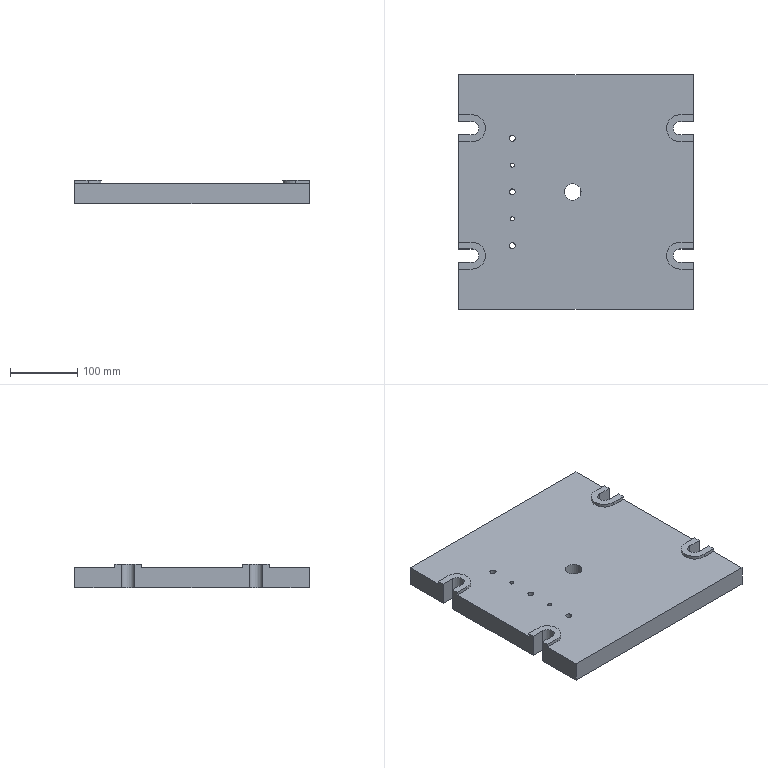Component | NX | FIXTURE_BASE | 1 solid | 50 faces | volume 3600373 mm3 | plane 33 | cylinder 17 | commonest cylinder face diameters 20 x4 40 x4 9 x3 15 x3 6 x2 25 x1